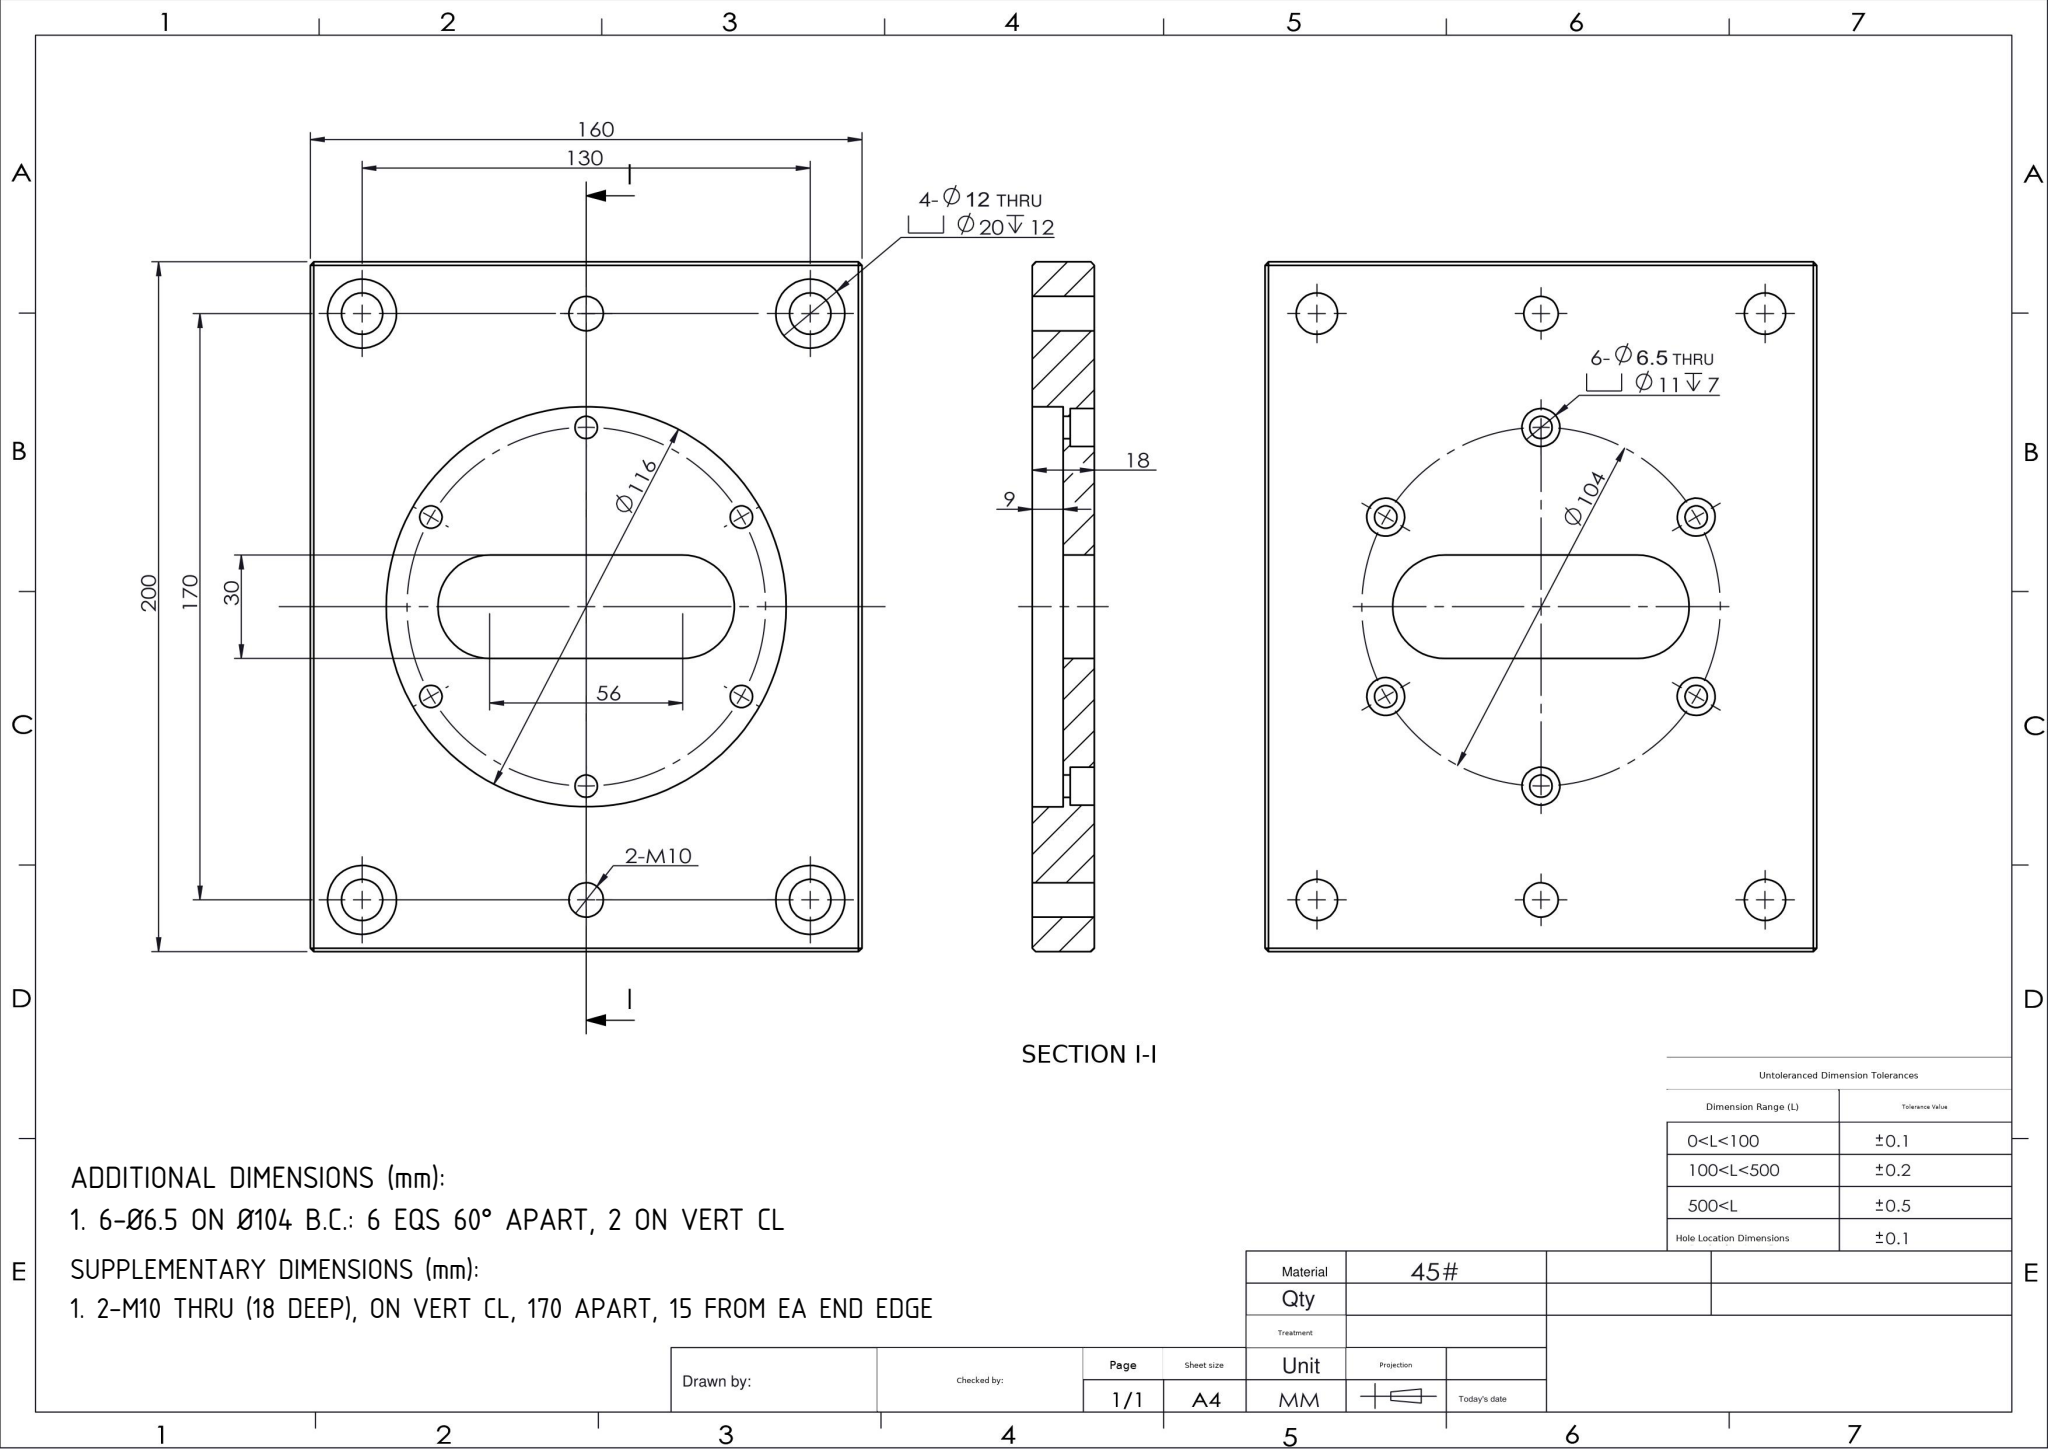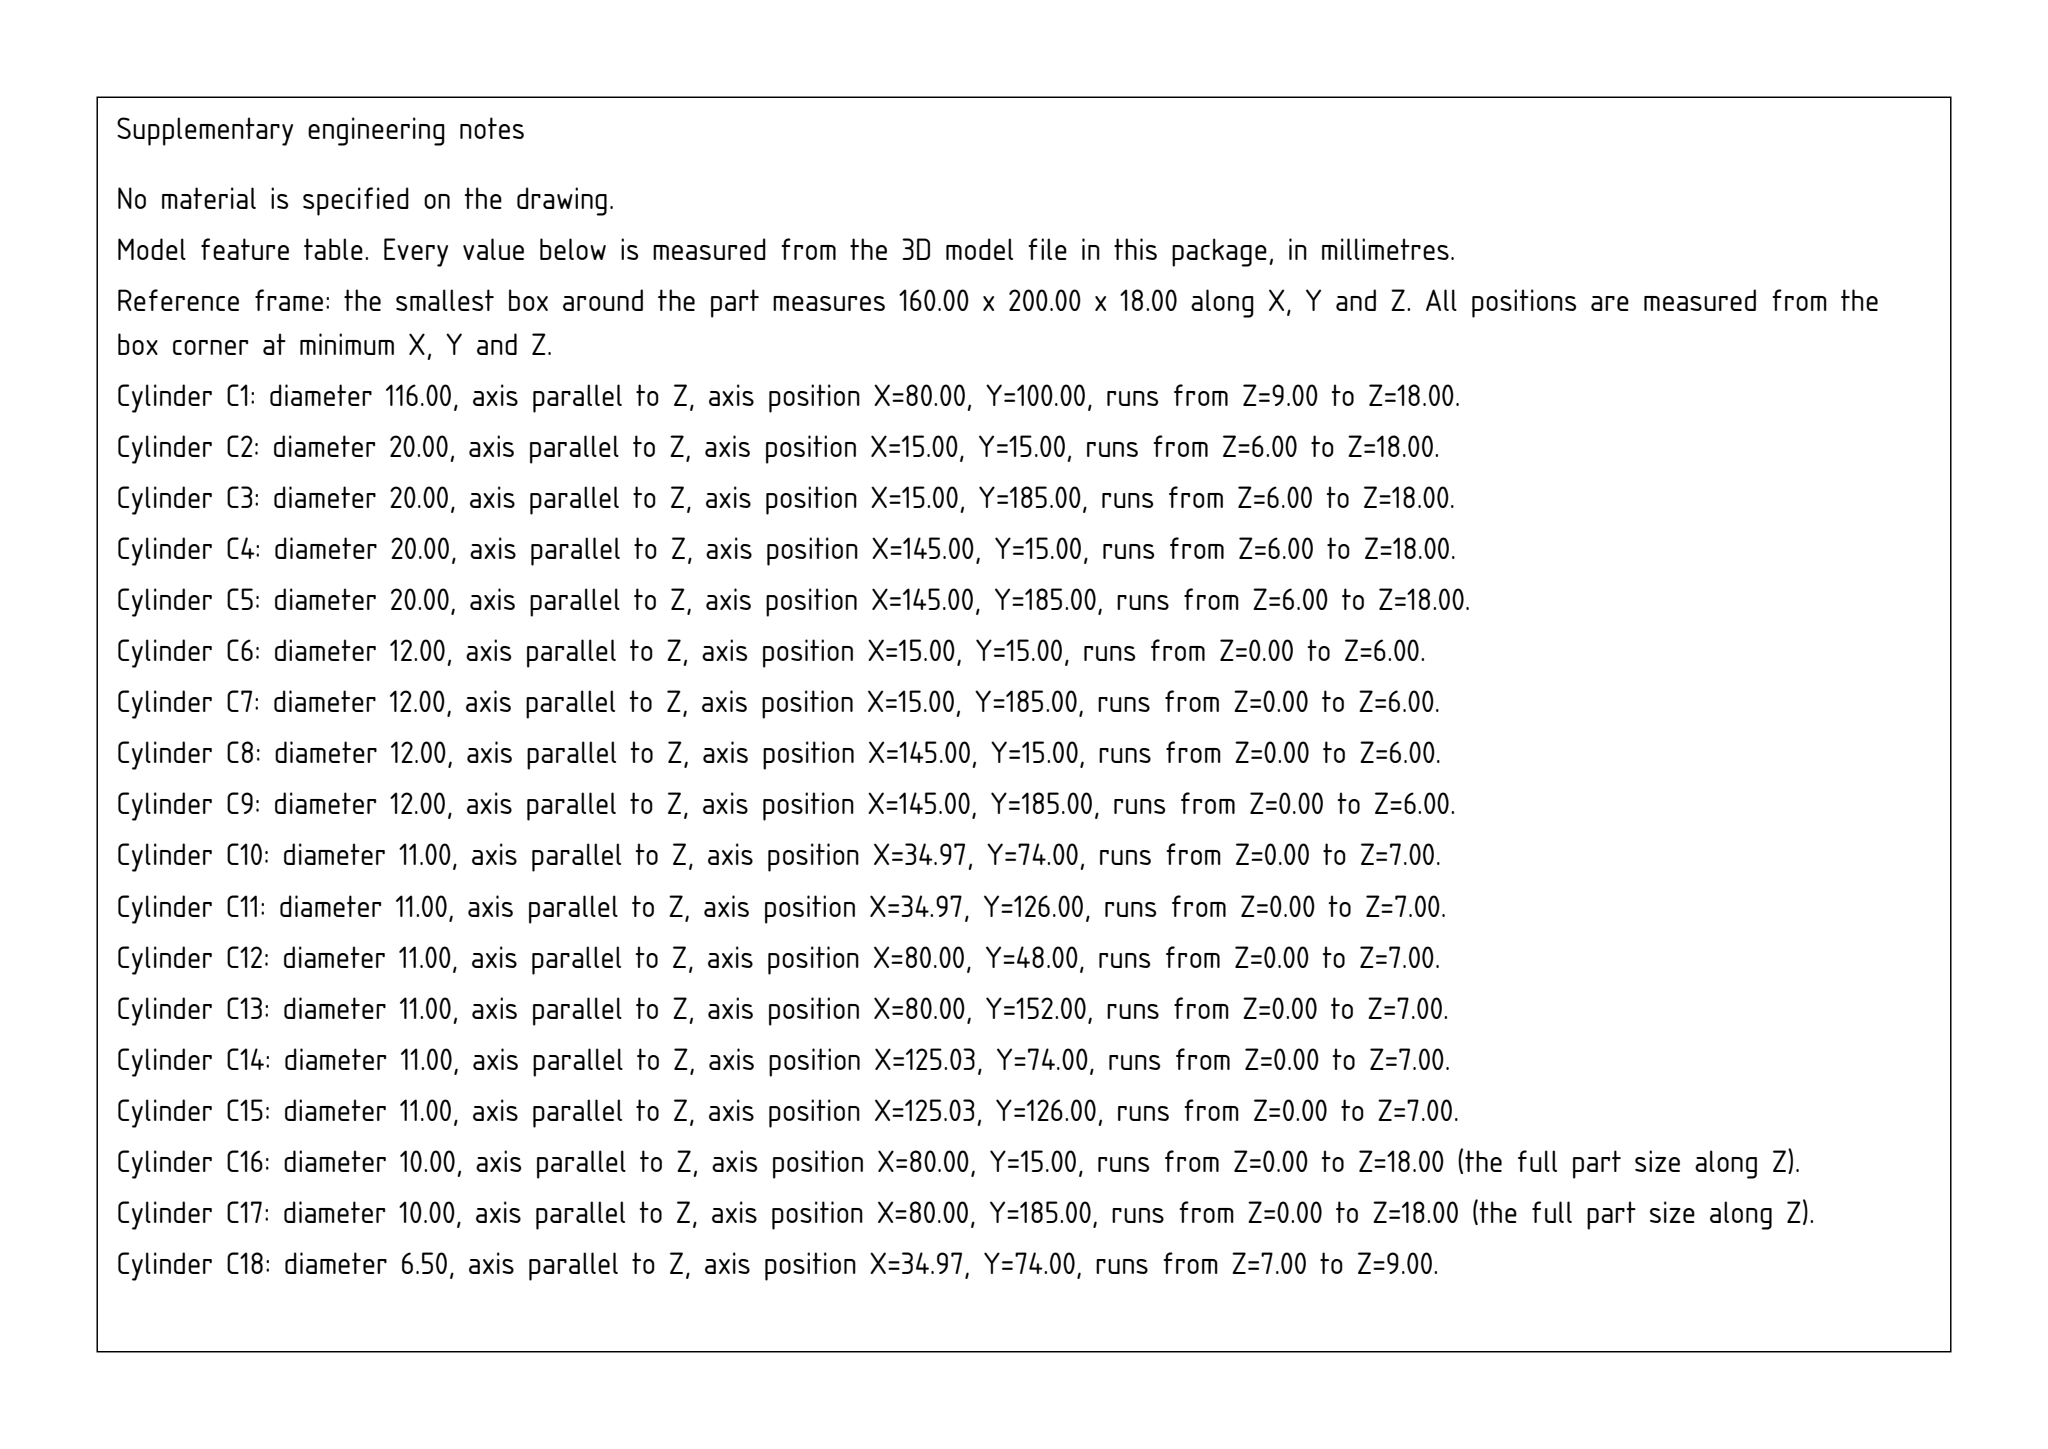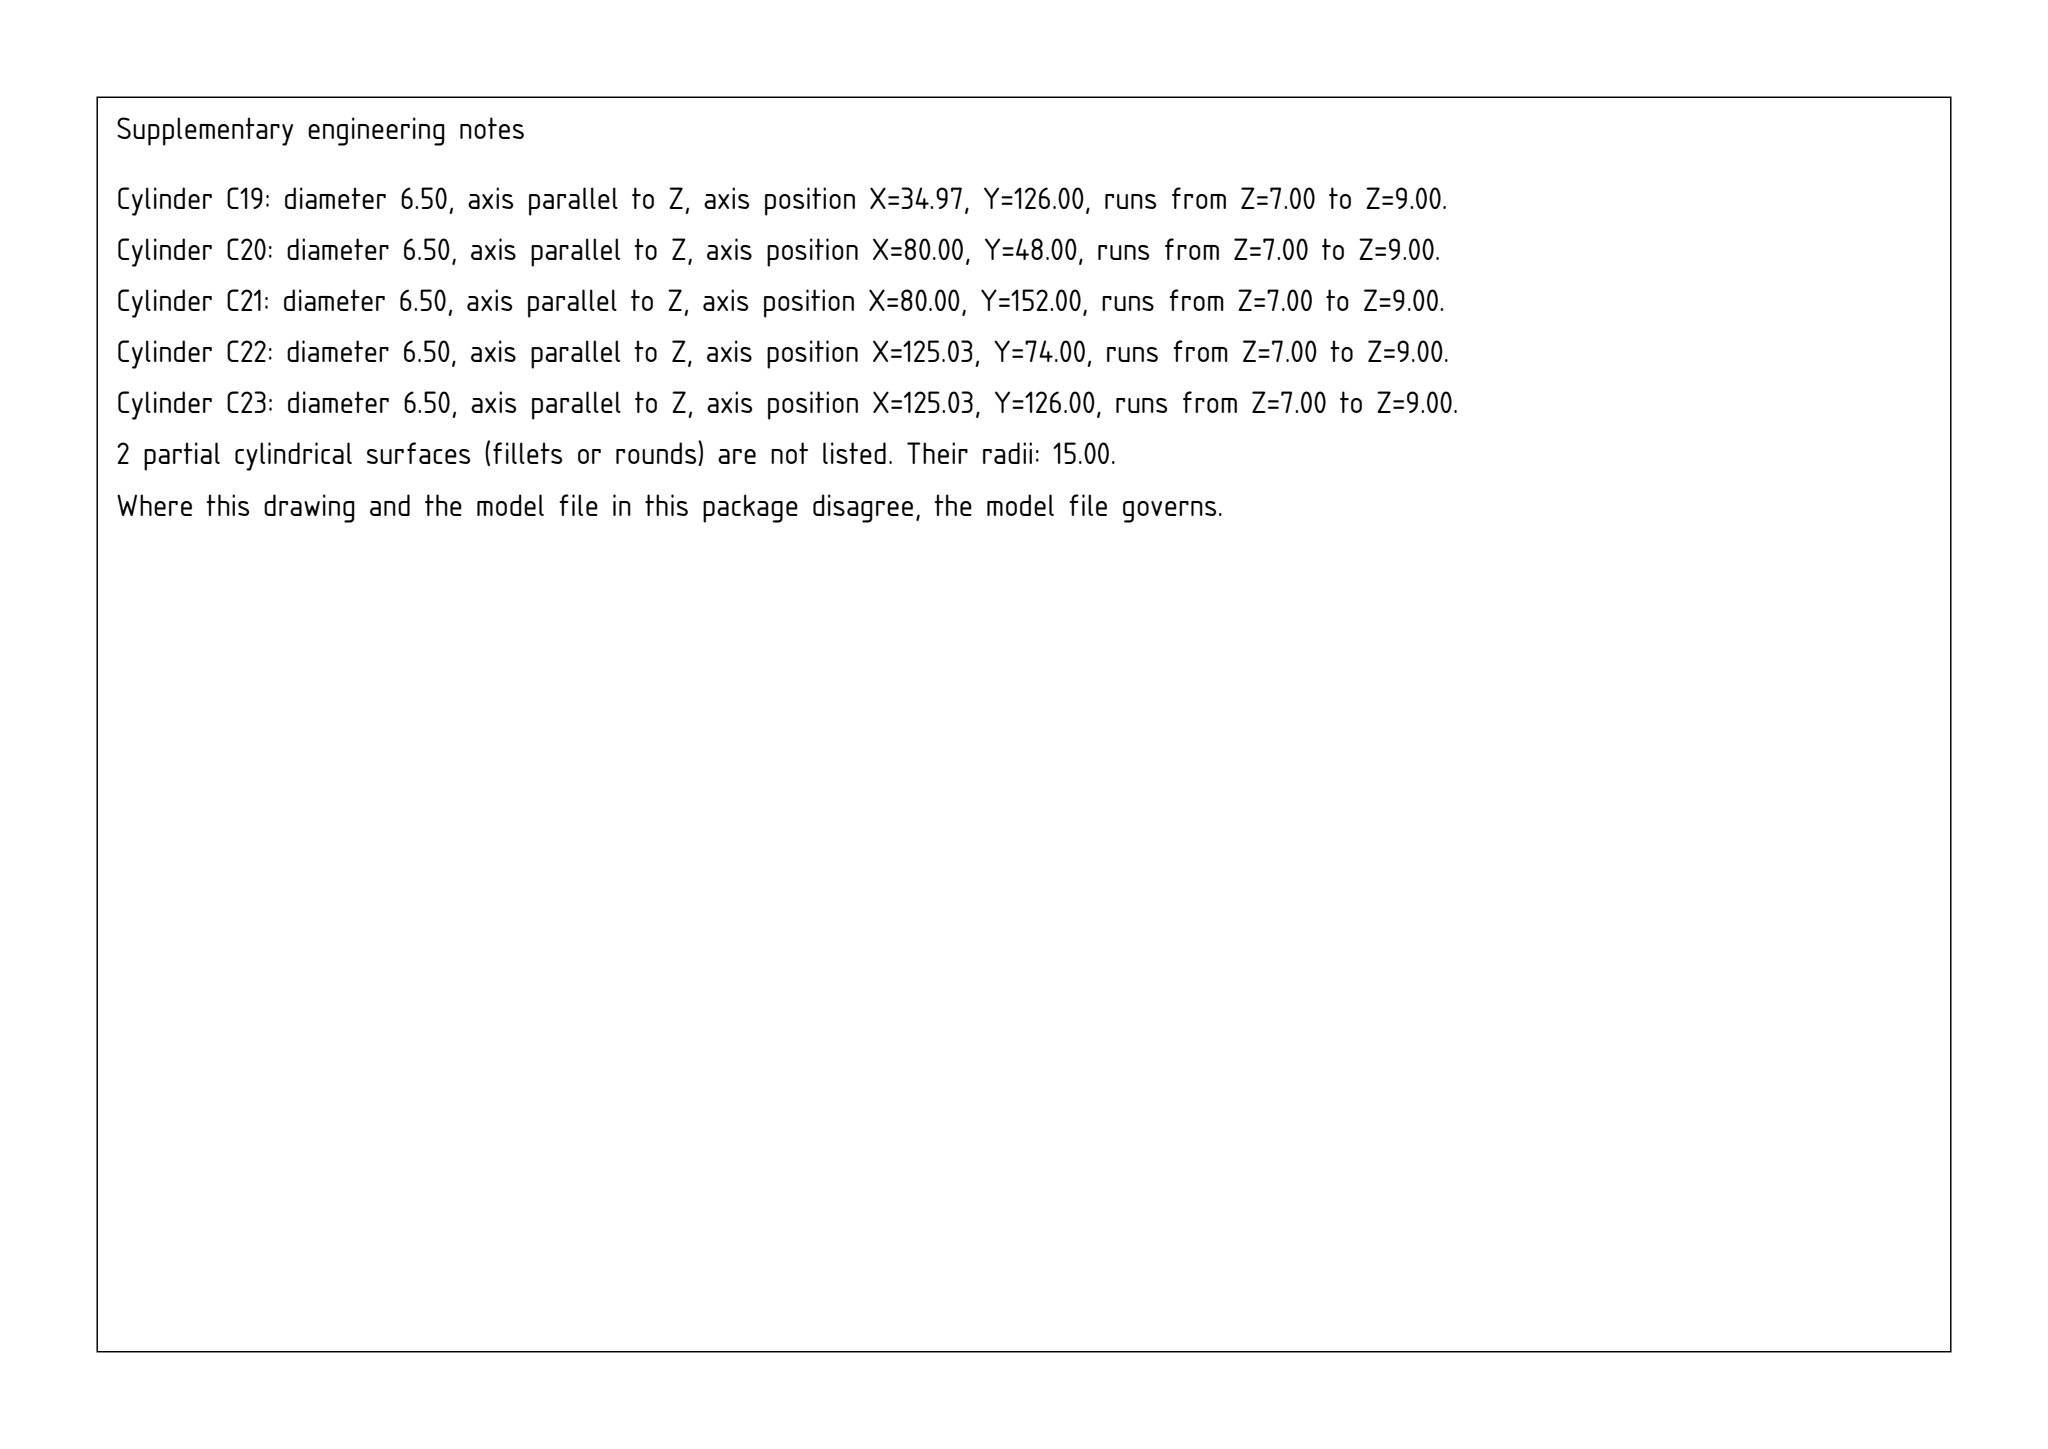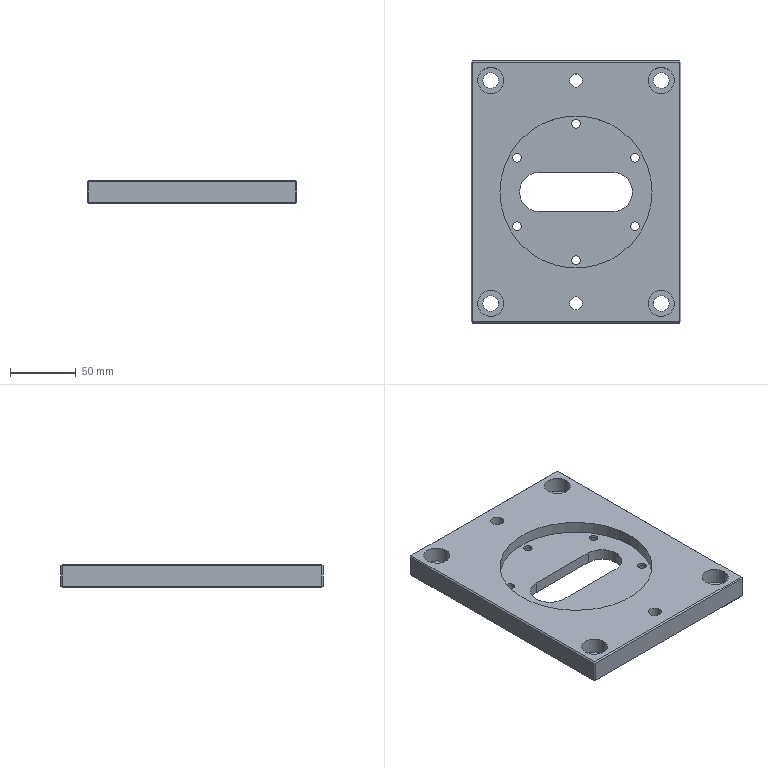Part | SolidWorks | mm | 1 solid | 88 faces | box 160 x 200 x 18 mm | volume 433642 mm3 | cylinder 49 | plane 39 | commonest cylinder face diameters 11 x12 6.5 x12 20 x8 12 x8 10 x4 30 x3 116 x2
build123d program:
from build123d import *

# Parameters (mm, degrees)
SKETCH1_W           = 160
SKETCH1_H           = 200
BOSS_EXTRUDE1_DEPTH = 9
SKETCH2_R           = 6
CUT_EXTRUDE1_DEPTH  = 130.321
SKETCH3_R           = 10
CUT_EXTRUDE2_DEPTH  = 12
CHAMFER1_SIZE       = 1
SKETCH4_R           = 58
CUT_EXTRUDE3_DEPTH  = 9
CUT_EXTRUDE4_DEPTH  = 130.321
SKETCH6_R           = 5
CUT_EXTRUDE5_DEPTH  = 130.321
SKETCH7_R           = 3.25
CUT_EXTRUDE6_DEPTH  = 130.321
SKETCH8_R           = 5.5
CUT_EXTRUDE7_DEPTH  = 7
CIRPATTERN1_COUNT   = 6


with BuildPart() as part:
    # Sketch1 → Boss-Extrude1 (new, symmetric)
    with BuildSketch(Plane.XY):
        Rectangle(SKETCH1_W, SKETCH1_H)
    extrude(amount=BOSS_EXTRUDE1_DEPTH, both=True)

    # Sketch2 → Cut-Extrude1 (cut, through all)
    with BuildSketch(Plane.XY.offset(9)):
        with Locations((-65, 85)):
            Circle(SKETCH2_R)
        with Locations(Location((65, 85, 0), (0, 0, 180))):
            Circle(SKETCH2_R)
        with Locations((65, -85)):
            Circle(SKETCH2_R)
        with Locations(Location((-65, -85, 0), (0, 0, 180))):
            Circle(SKETCH2_R)
    extrude(amount=-CUT_EXTRUDE1_DEPTH, mode=Mode.SUBTRACT)

    # Sketch3 → Cut-Extrude2 (cut)
    with BuildSketch(Plane.XY.offset(9)):
        with Locations((-65, 85)):
            Circle(SKETCH3_R)
        with Locations((65, 85)):
            Circle(SKETCH3_R)
        with Locations((-65, -85)):
            Circle(SKETCH3_R)
        with Locations((65, -85)):
            Circle(SKETCH3_R)
    extrude(amount=-CUT_EXTRUDE2_DEPTH, mode=Mode.SUBTRACT)

    # Chamfer1
    chamfer1_edges = [part.edges().sort_by_distance(p)[0] for p in [
        (-80, 0, 9),
        (0, -100, 9),
        (80, 0, 9),
        (0, -100, -9),
        (-80, 0, -9),
        (0, 100, -9),
        (80, 0, -9),
        (0, 100, 9),
        (80, -100, 0),
        (-80, -100, 0),
        (-80, 100, 0),
        (80, 100, 0),
    ]]
    chamfer(chamfer1_edges, length=CHAMFER1_SIZE)

    # Sketch4 → Cut-Extrude3 (cut)
    with BuildSketch(Plane.XY.offset(9)):
        Circle(SKETCH4_R)
    extrude(amount=-CUT_EXTRUDE3_DEPTH, mode=Mode.SUBTRACT)

    # Sketch5 → Cut-Extrude4 (cut, through all)
    with BuildSketch(Plane.XY.offset(9)):
        with BuildLine():
            Line((-28, 15), (28, 15))
            ThreePointArc((28, 15), (43, 0), (28, -15))
            Line((28, -15), (-28, -15))
            ThreePointArc((-28, -15), (-43, 0), (-28, 15))
        make_face()
    extrude(amount=-CUT_EXTRUDE4_DEPTH, mode=Mode.SUBTRACT)

    # Sketch6 → Cut-Extrude5 (cut, through all)
    with BuildSketch(Plane.XY.offset(9)):
        with Locations((0, 85)):
            Circle(SKETCH6_R)
        with Locations(Location((0, -85, 0), (0, 0, 180))):
            Circle(SKETCH6_R)
    extrude(amount=-CUT_EXTRUDE5_DEPTH, mode=Mode.SUBTRACT)

    # Sketch7 → Cut-Extrude6 (cut, through all)
    with BuildSketch(Plane.XY.offset(9)):
        with Locations((0, 52)):
            Circle(SKETCH7_R)
    cut_extrude6 = extrude(amount=-CUT_EXTRUDE6_DEPTH, mode=Mode.SUBTRACT)

    # Sketch8 → Cut-Extrude7 (cut)
    with BuildSketch(Plane(origin=(0, 0, -9), x_dir=(-1, 0, 0), z_dir=(0, 0, -1))):
        with Locations((0, 52)):
            Circle(SKETCH8_R)
    cut_extrude7 = extrude(amount=-CUT_EXTRUDE7_DEPTH, mode=Mode.SUBTRACT)

    # CirPattern1: Cut-Extrude6, Cut-Extrude7 ×6 about axis
    cirpattern1_axis = Axis((0, 0, 0), (0, 0, 1))
    add([cut_extrude6.rotate(cirpattern1_axis, i * 360 / CIRPATTERN1_COUNT) for i in range(1, CIRPATTERN1_COUNT)], mode=Mode.SUBTRACT)
    add([cut_extrude7.rotate(cirpattern1_axis, i * 360 / CIRPATTERN1_COUNT) for i in range(1, CIRPATTERN1_COUNT)], mode=Mode.SUBTRACT)


solid = part.part